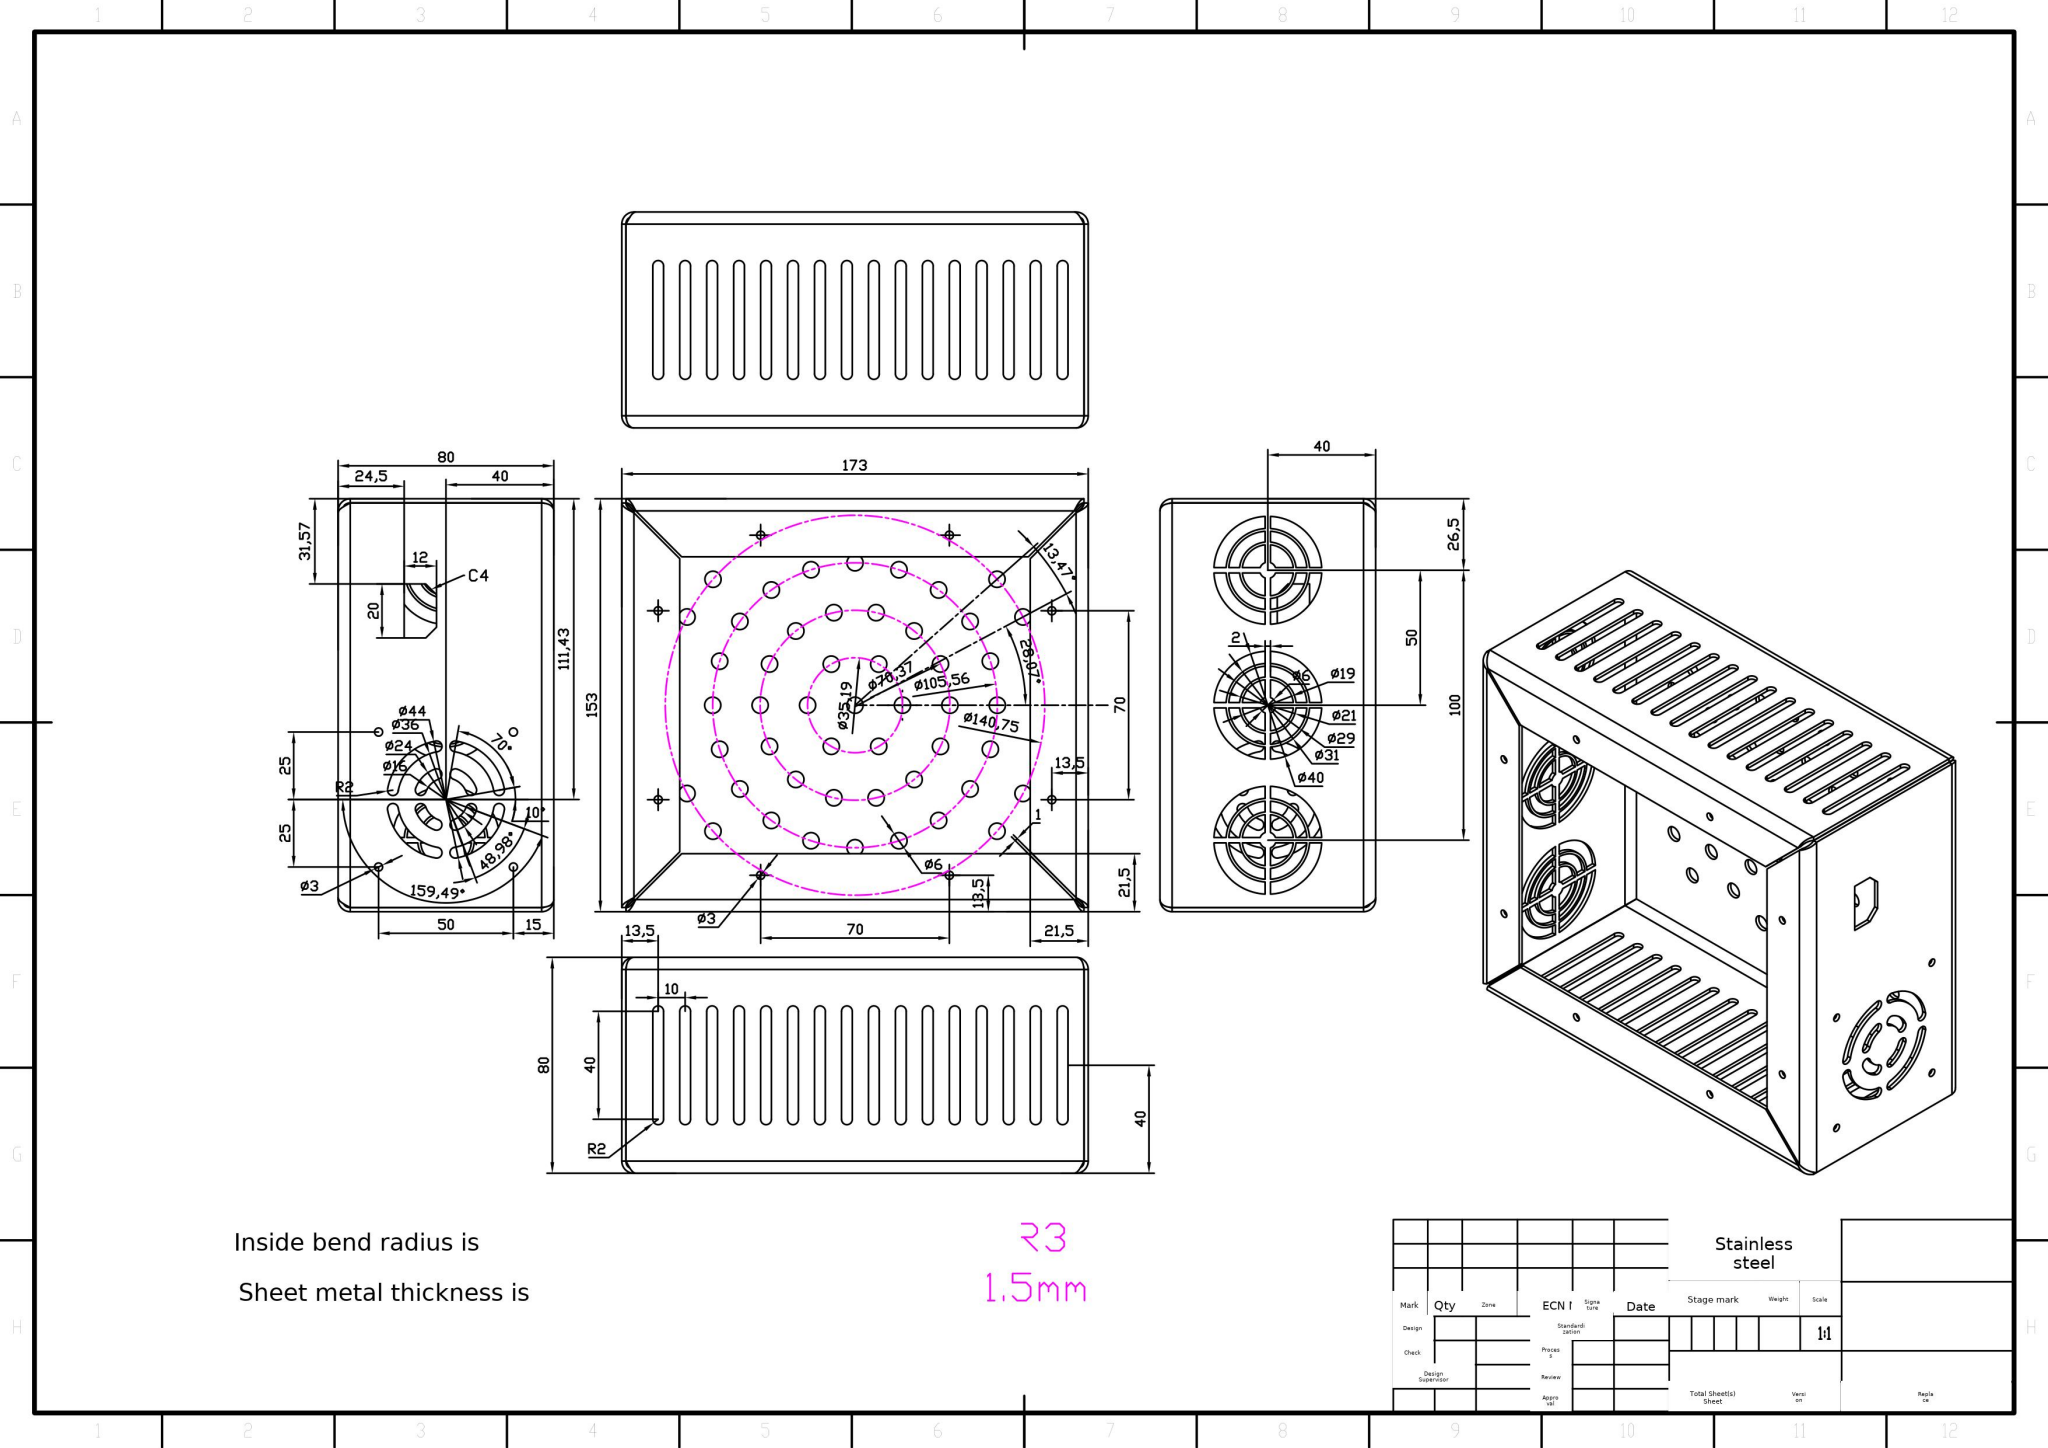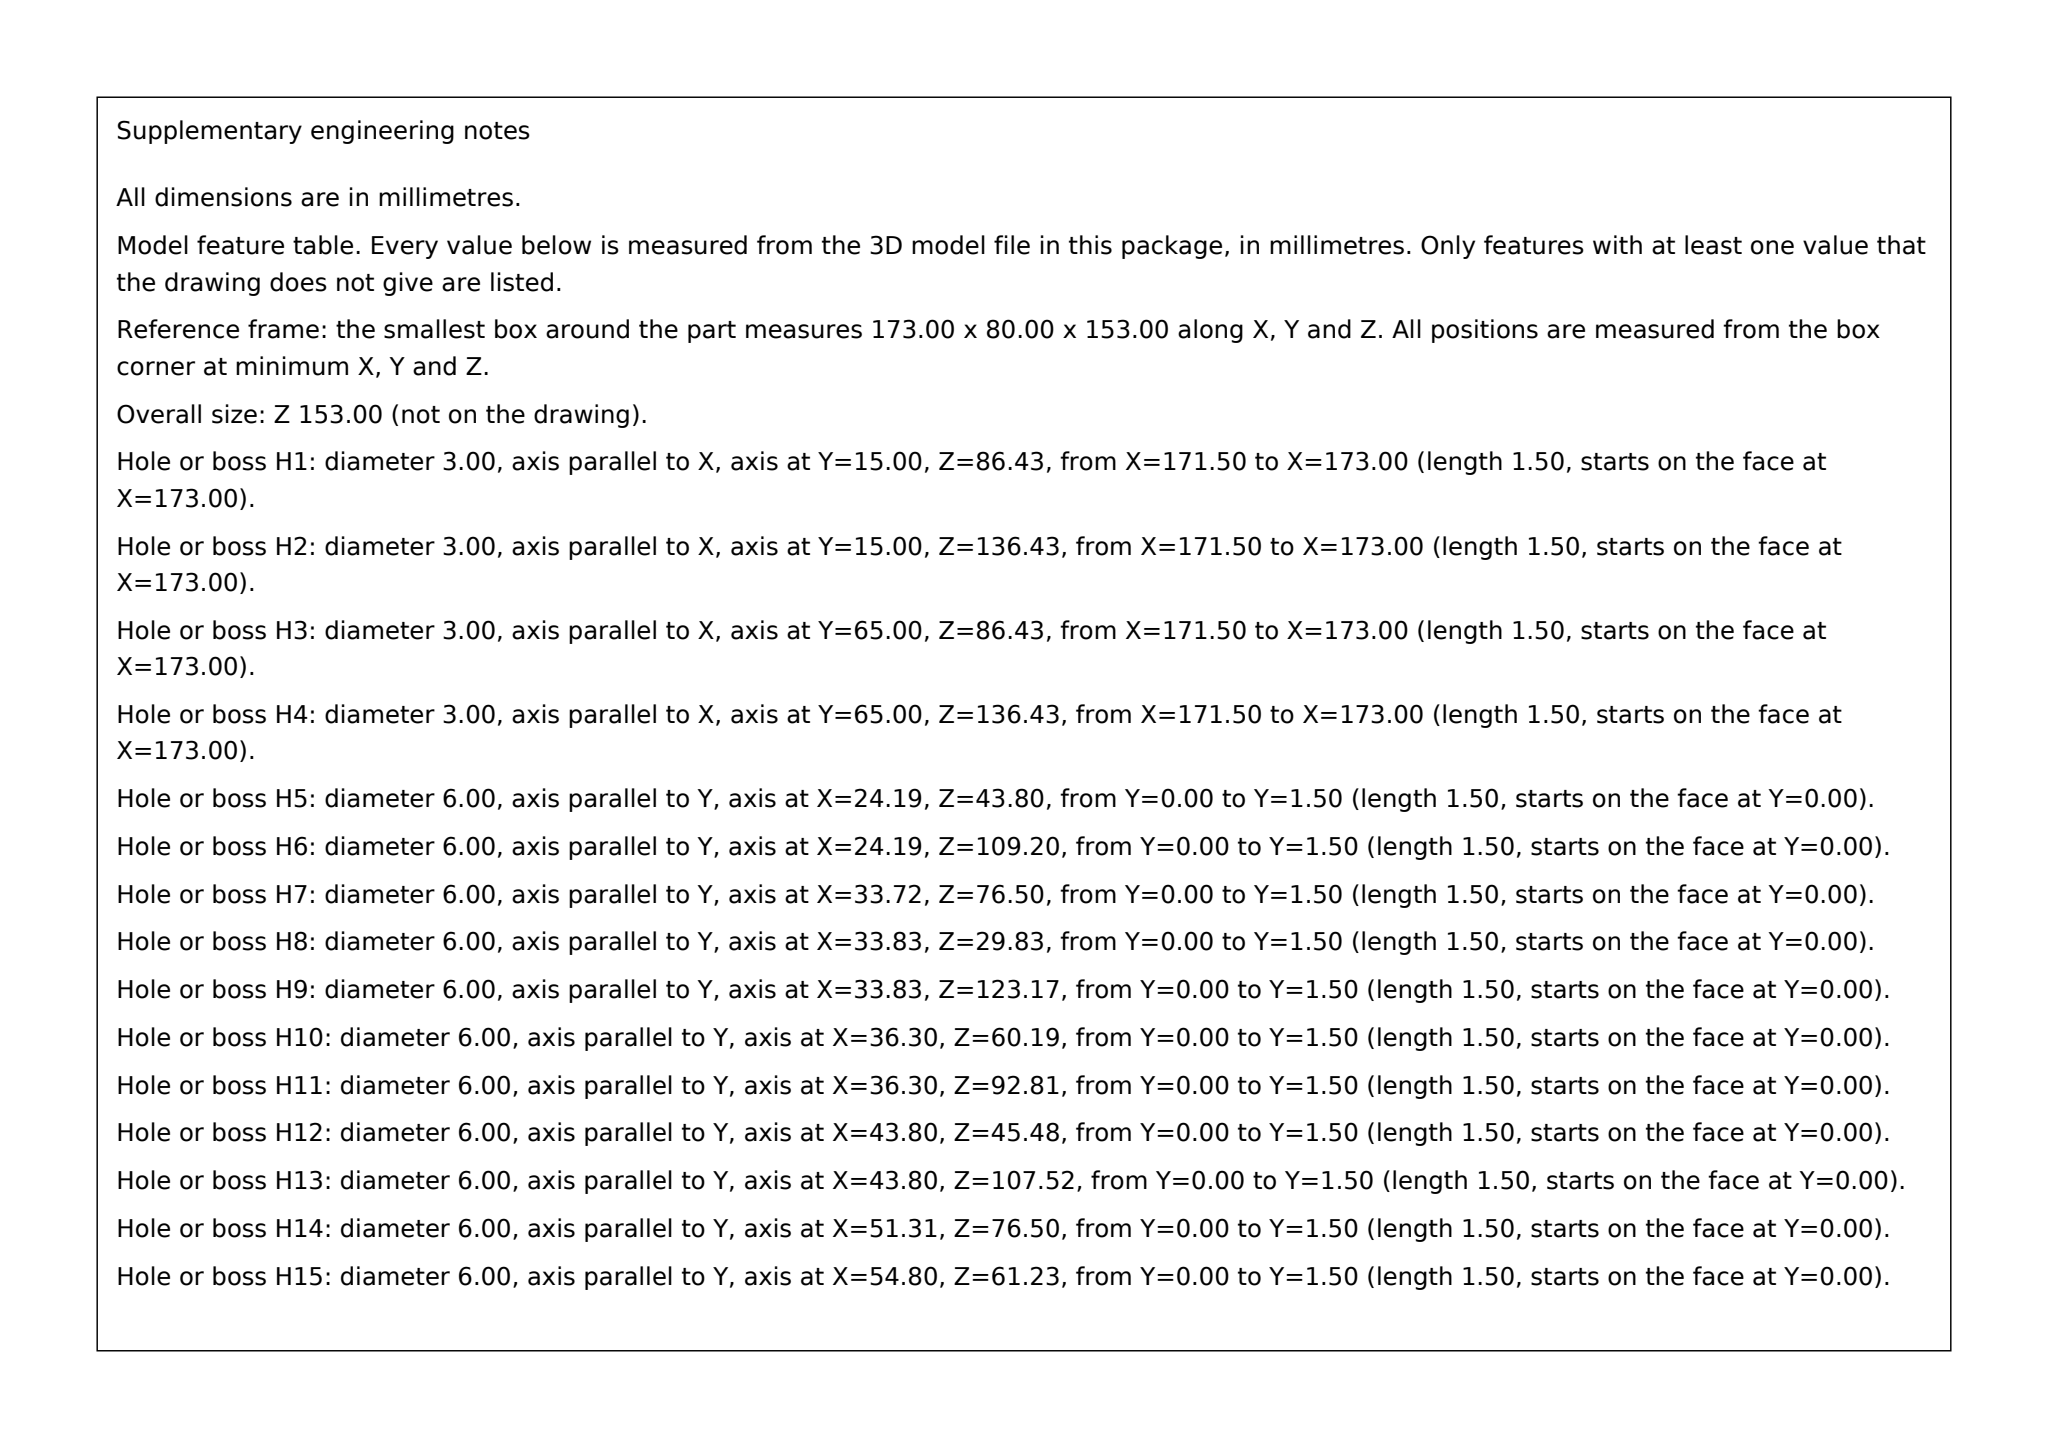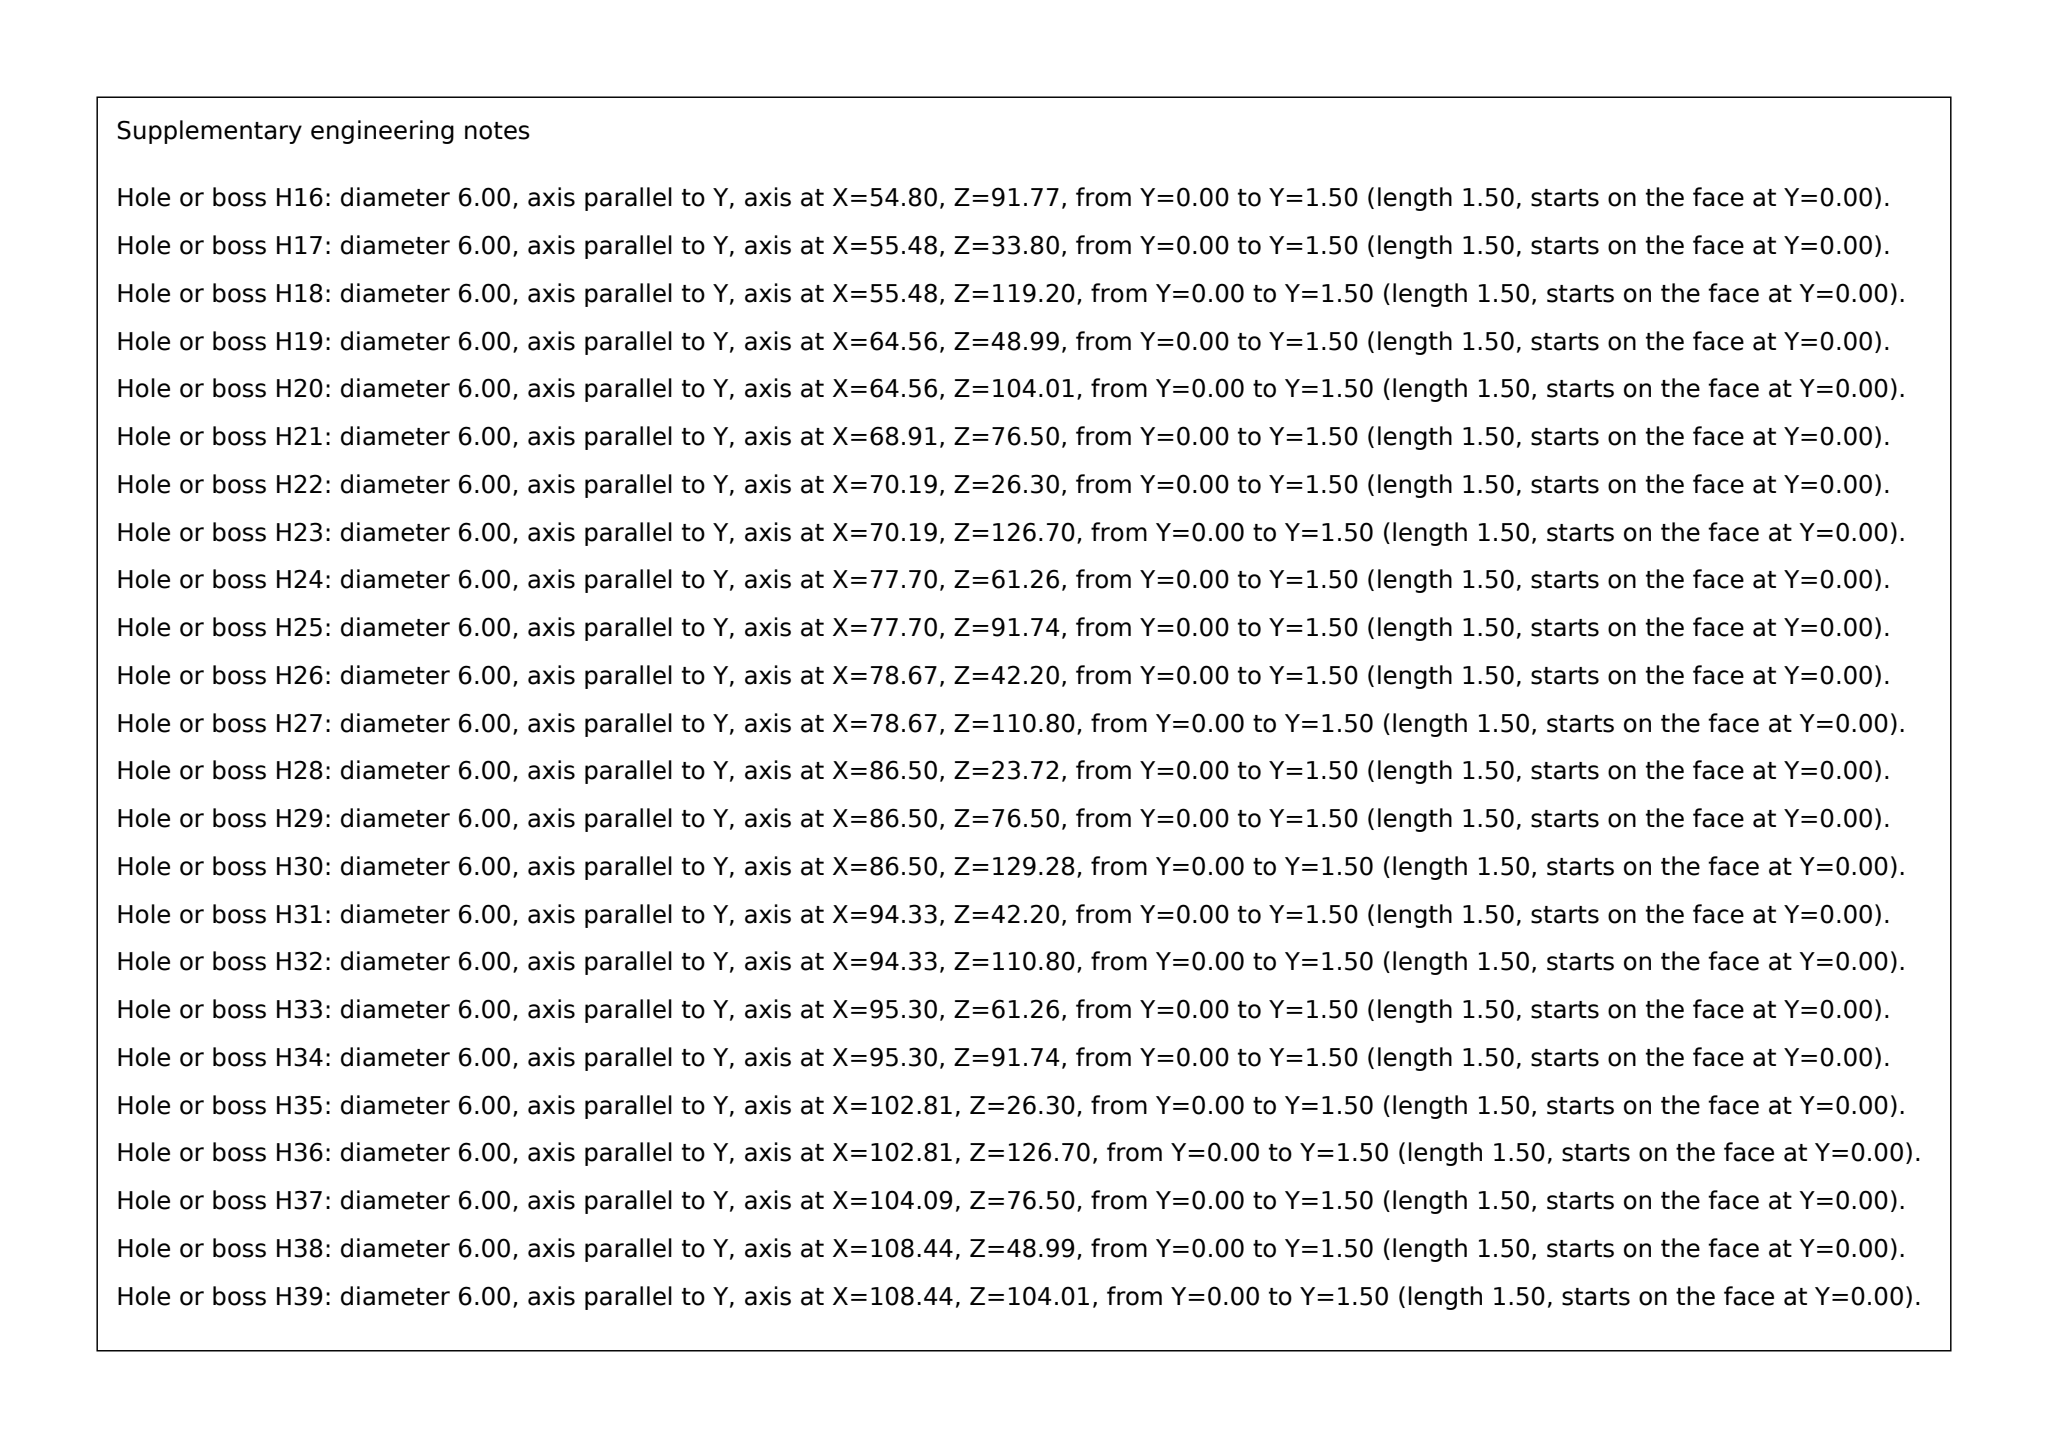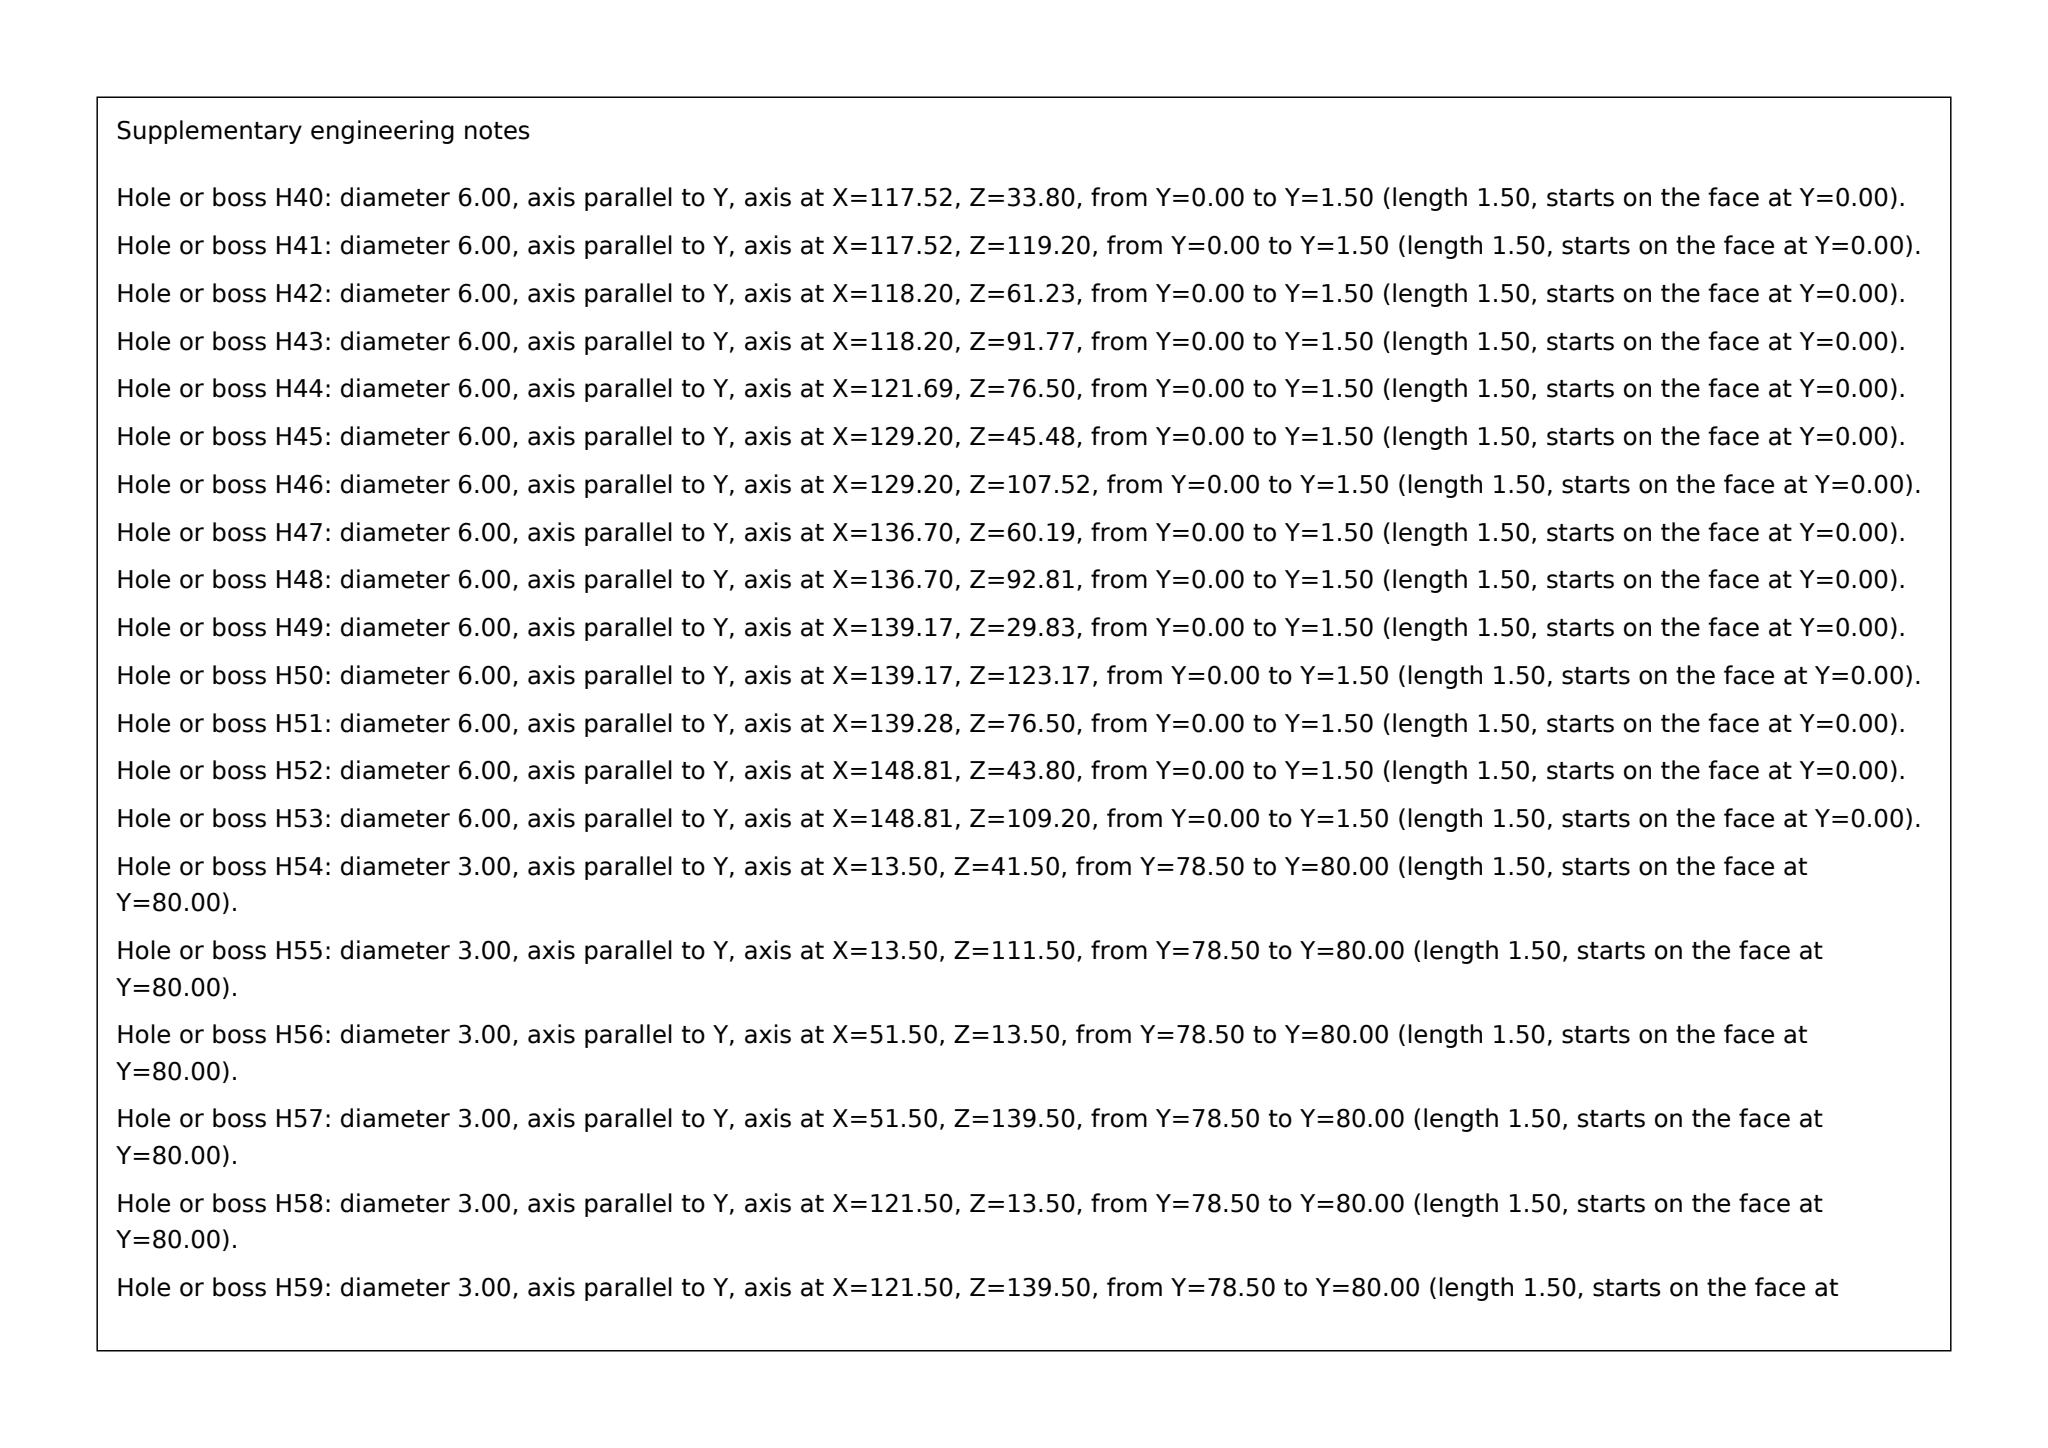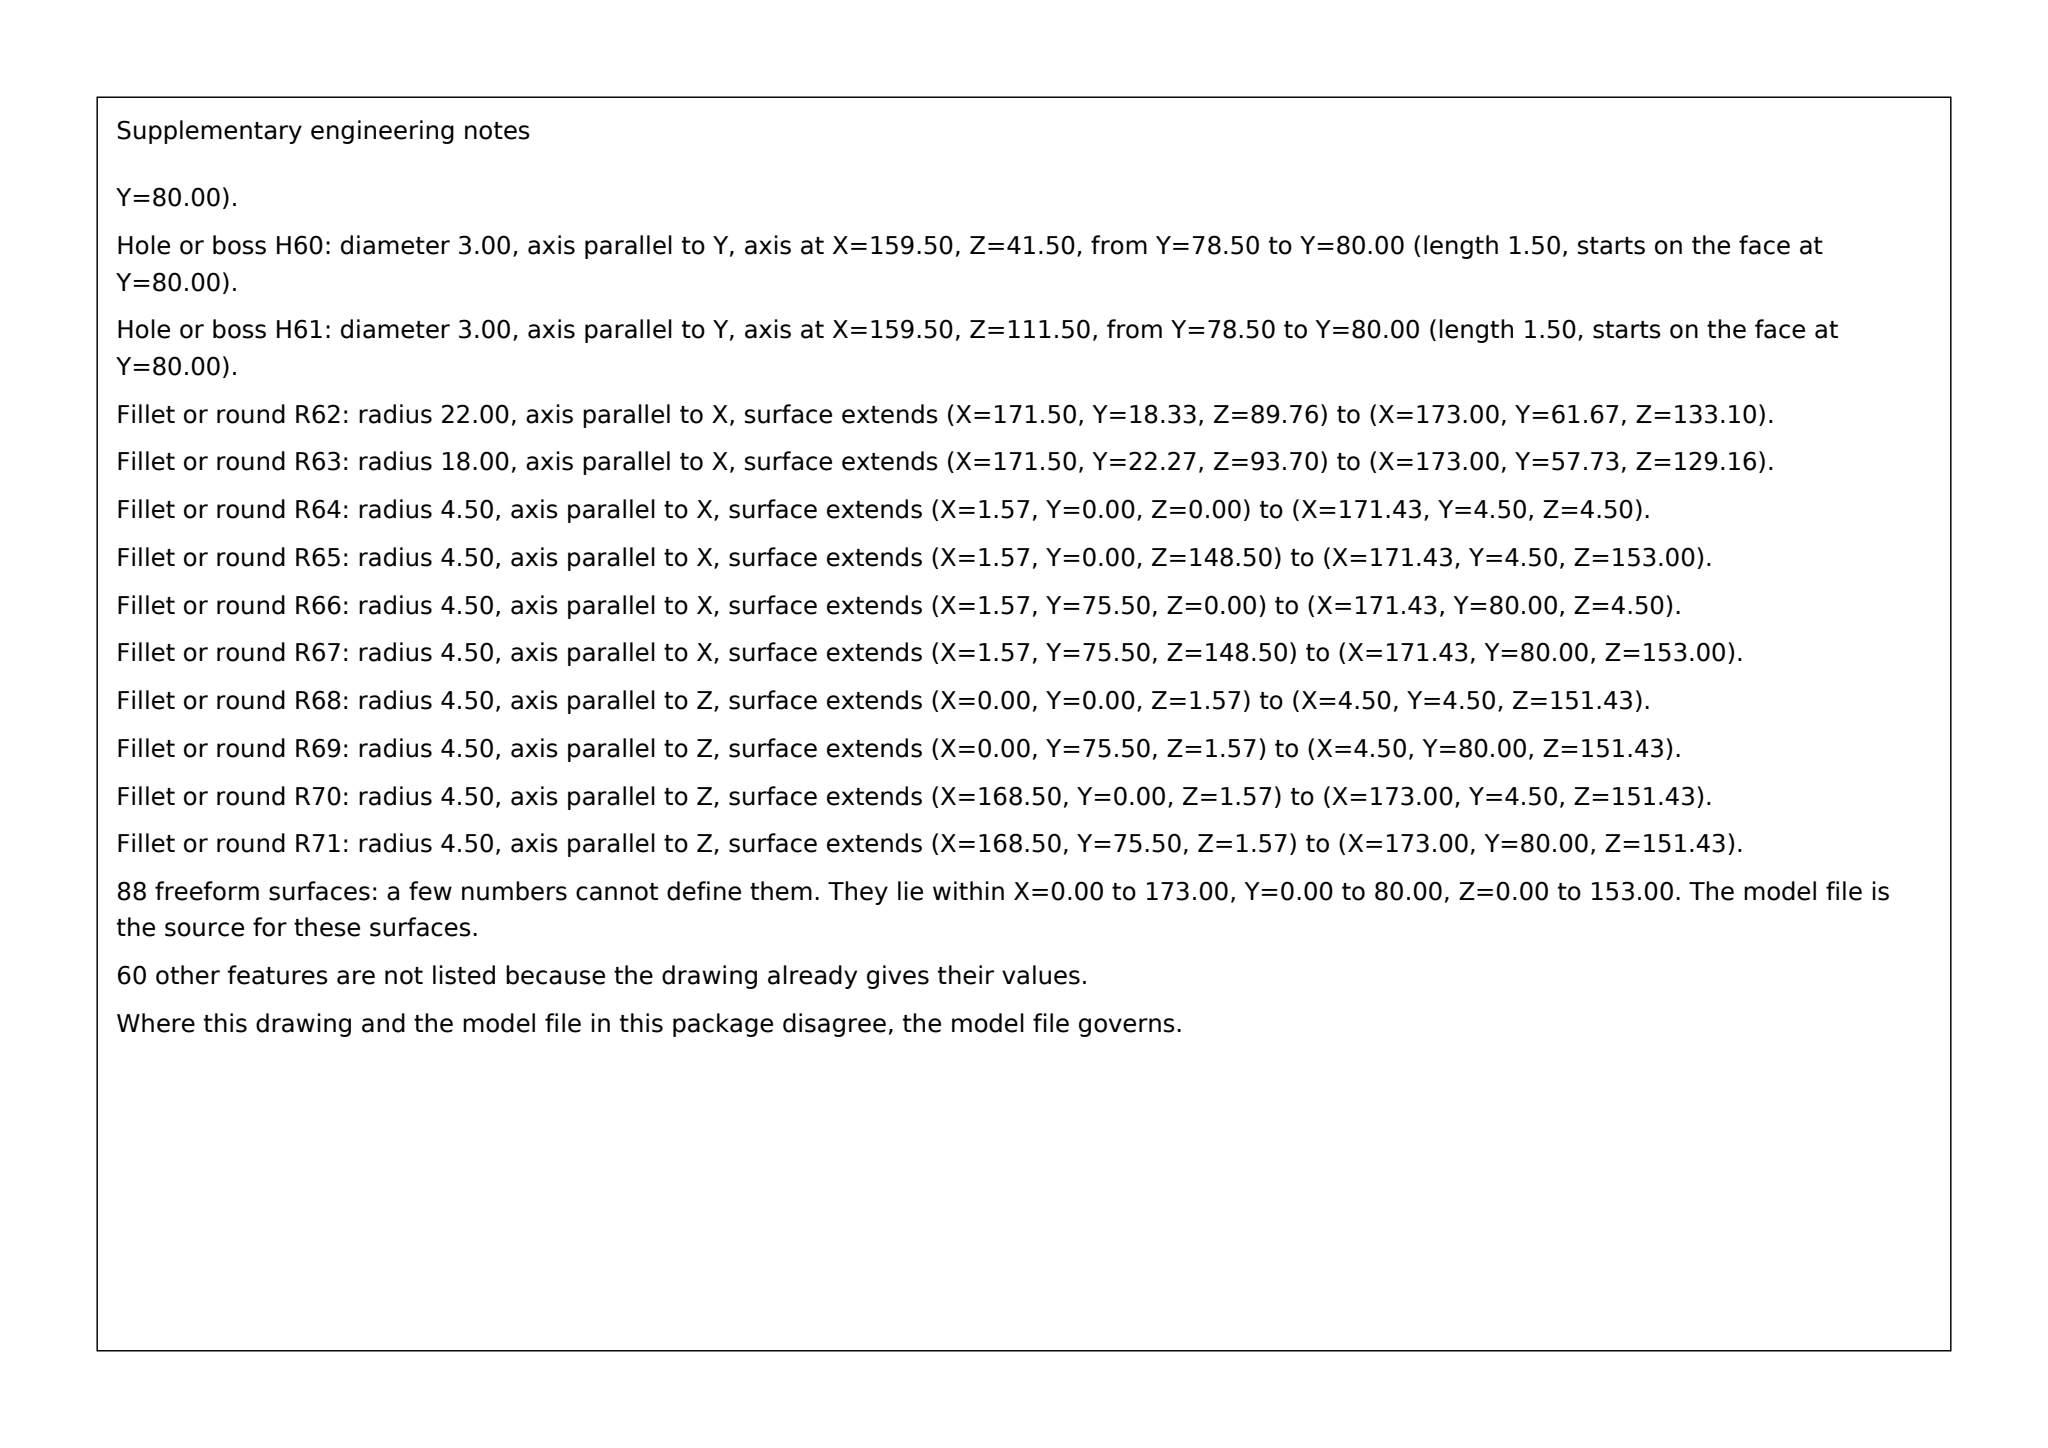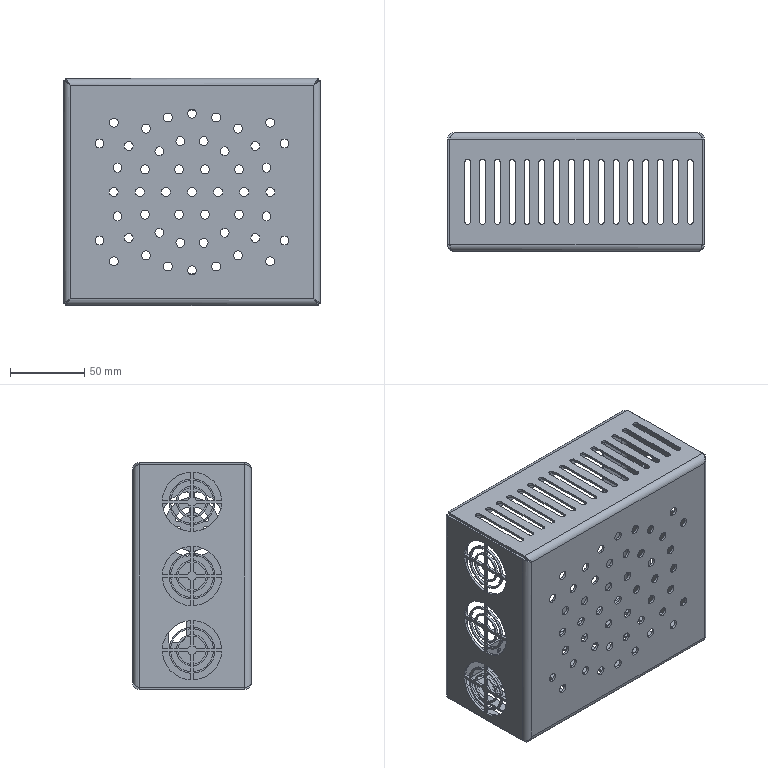Part | SolidWorks | mm | material Stainless steel | 1 solid | 510 faces | box 173 x 80 x 153 mm | volume 112402 mm3 | cylinder 242 | plane 180 | spline 88 | commonest cylinder face diameters 6 x106 4 x88 3 x24 9 x8 44 x4 36 x4 16 x4 24 x4